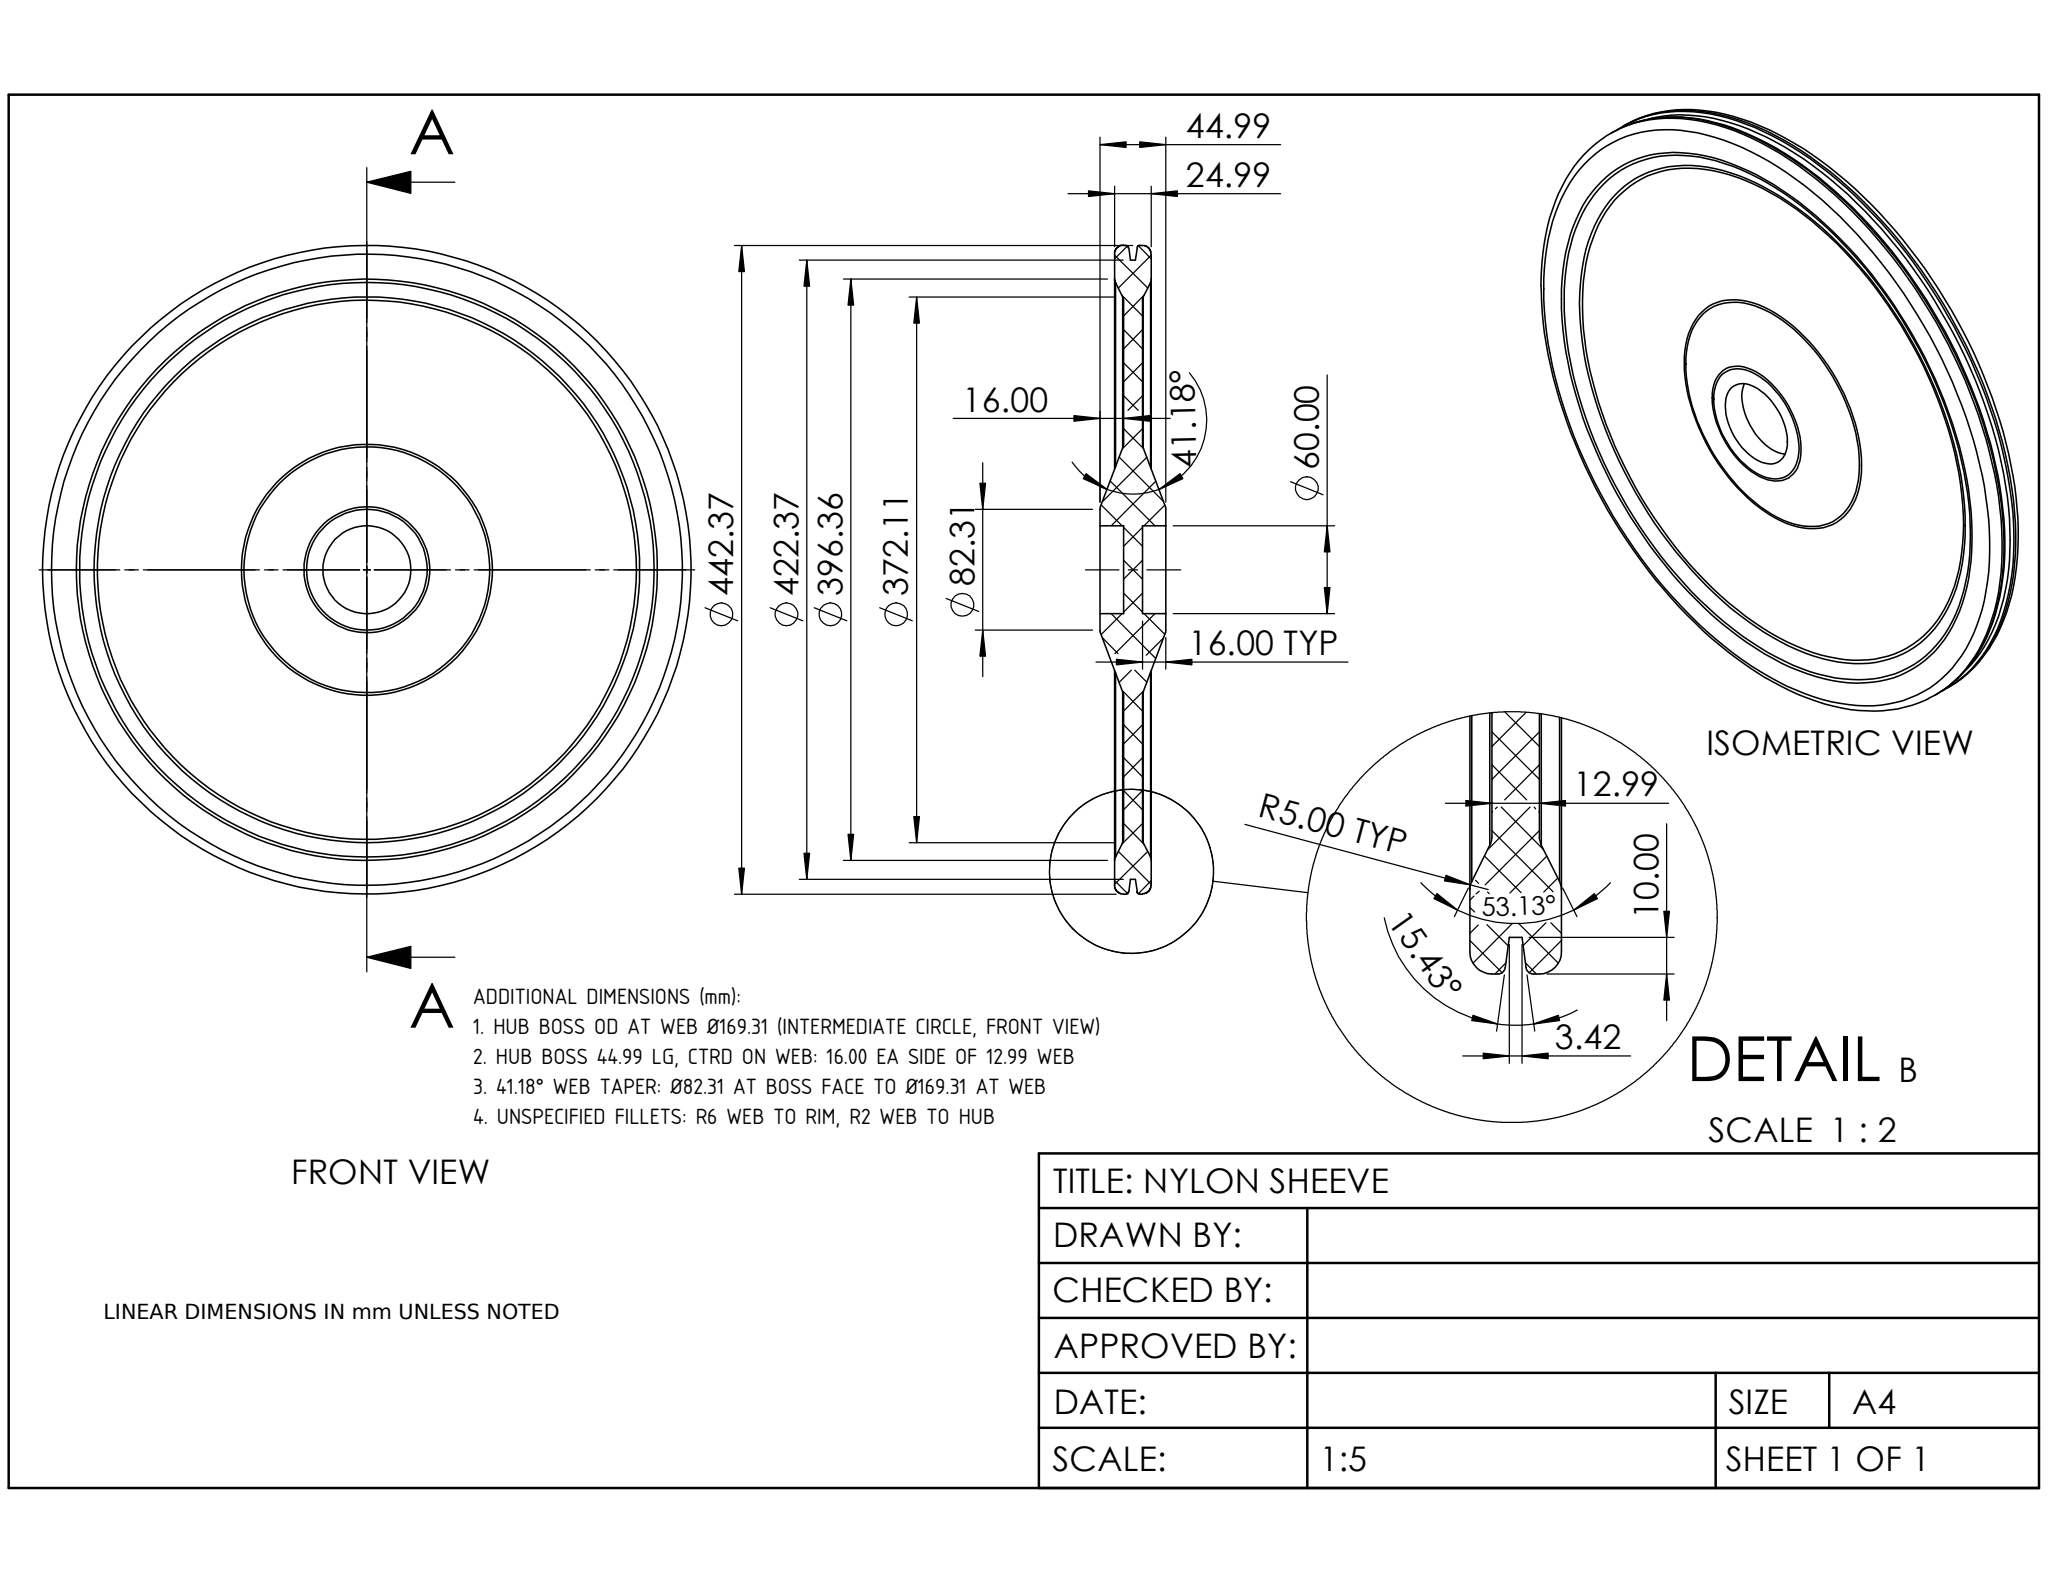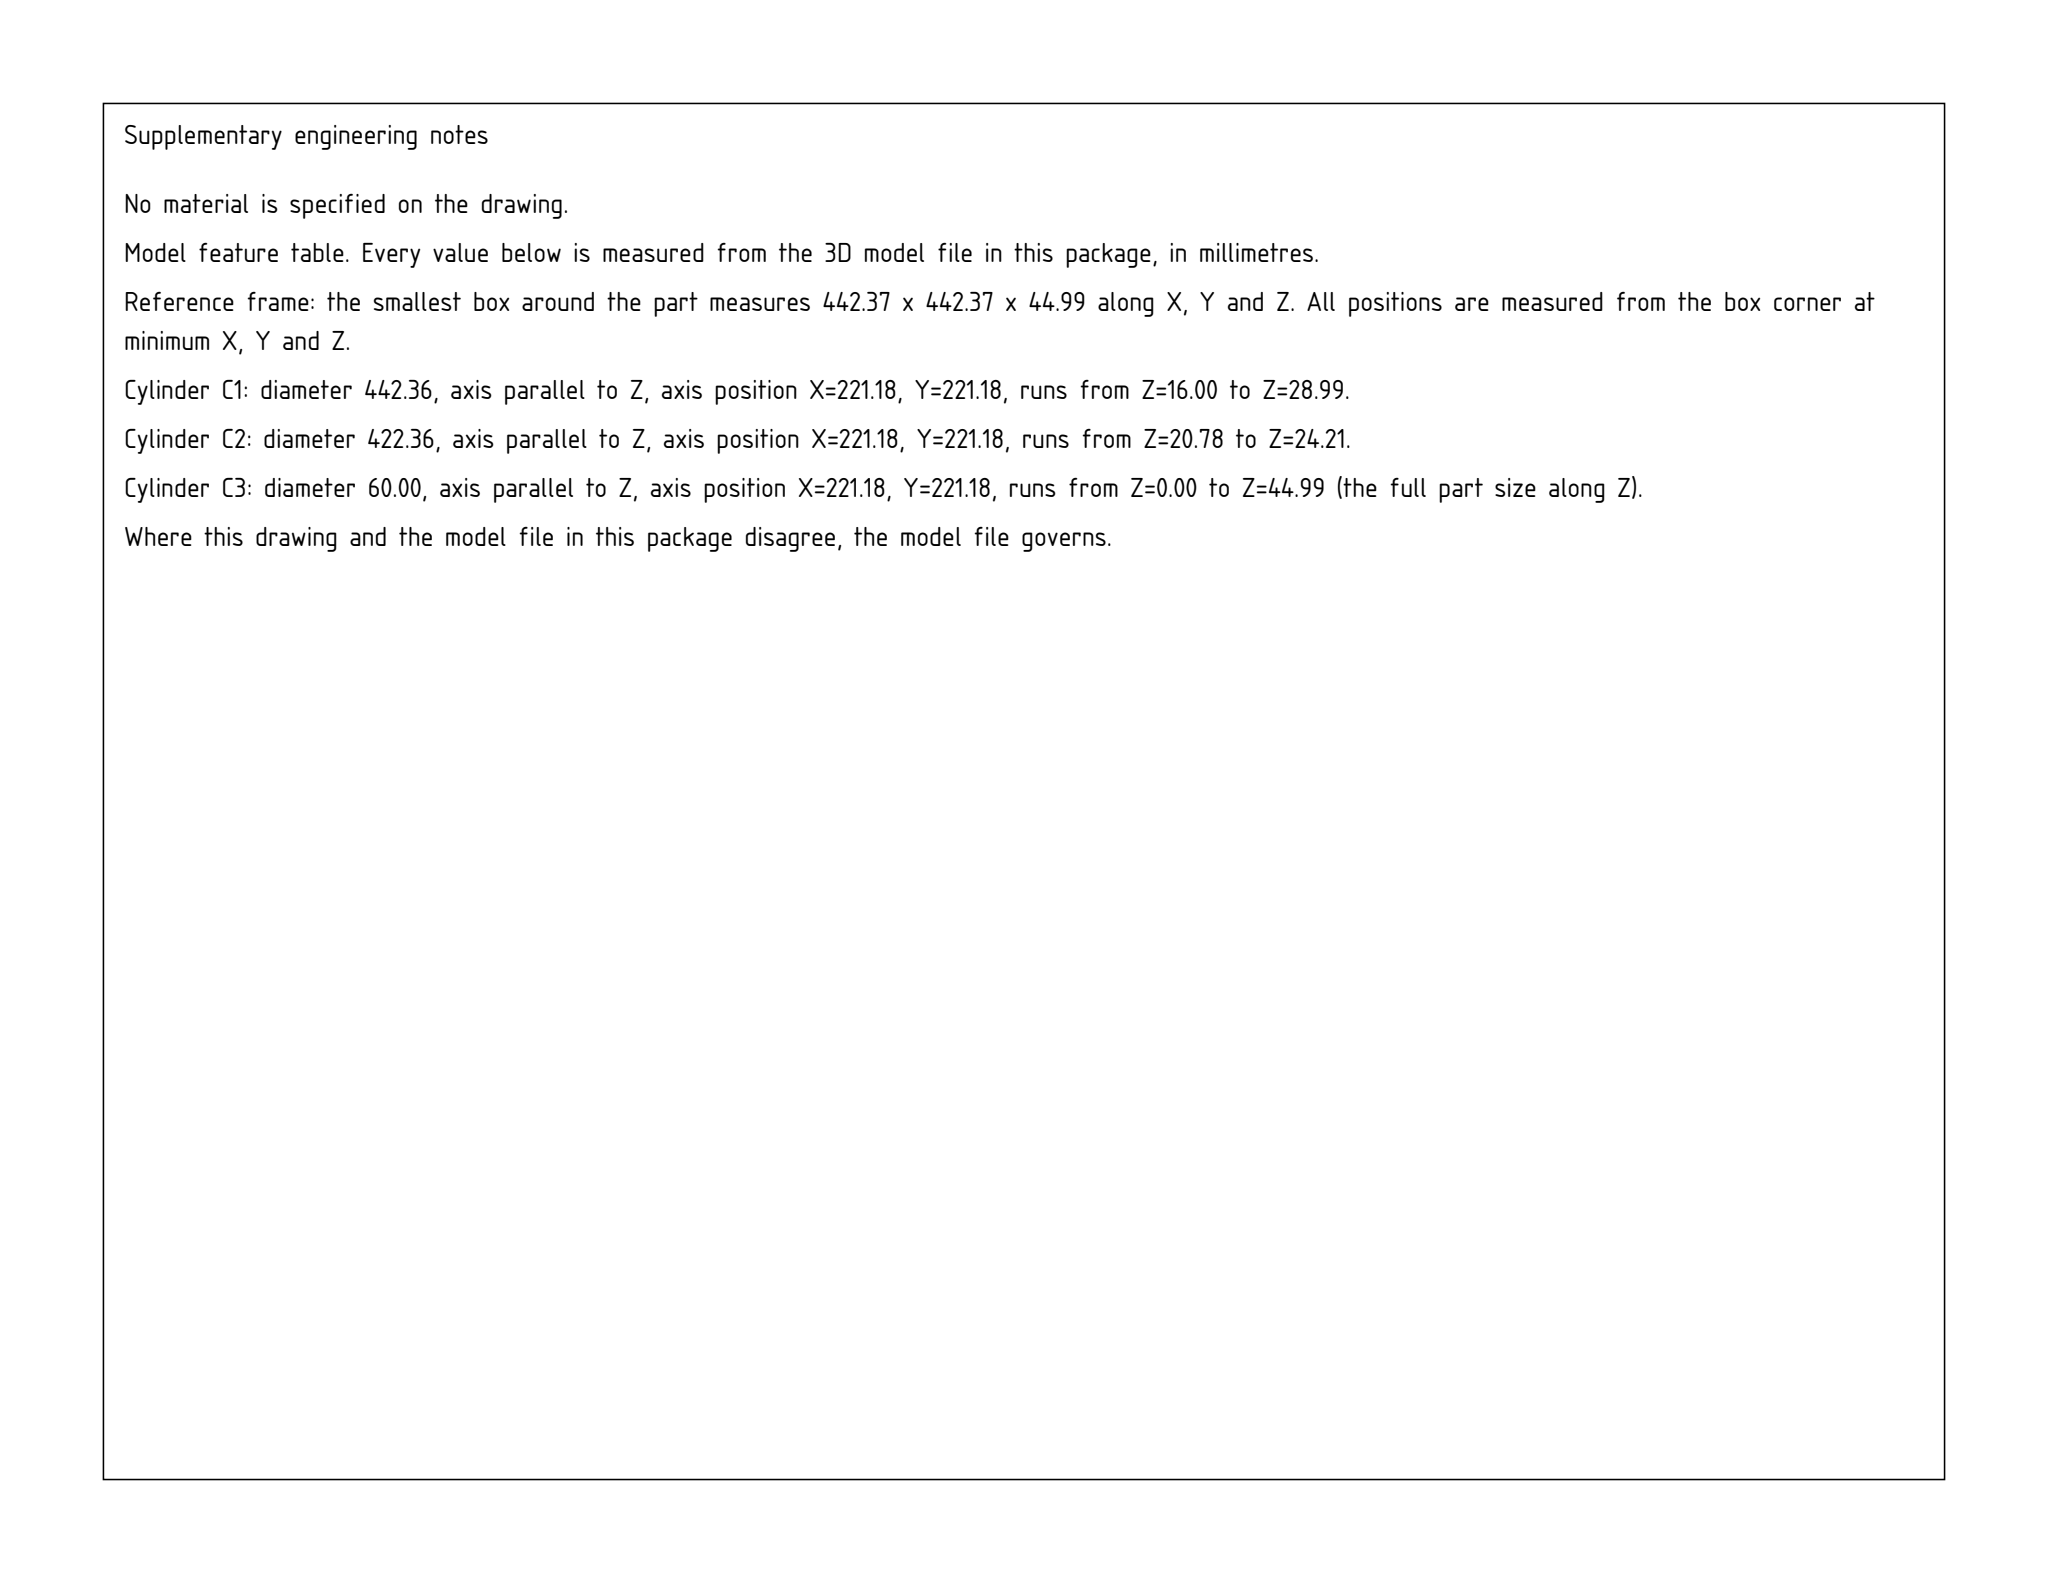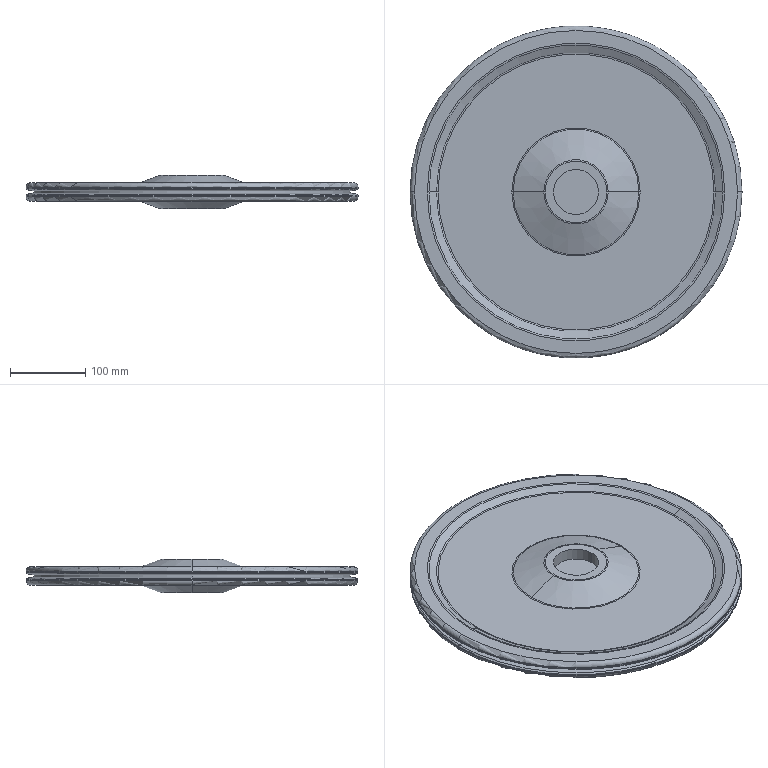Part | SolidWorks | mm | 1 solid | 54 faces | box 442.37 x 442.37 x 44.99 mm | volume 2705251 mm3 | torus 24 | cone 12 | cylinder 10 | plane 8 | commonest cylinder face diameters 60 x4 442.365 x4 422.365 x2
build123d program:
from build123d import *

# Parameters (mm, degrees)
FILLET1_R          = 6
FILLET2_R          = 2
FILLET4_R          = 5
SKETCH3_R          = 30
CUT_EXTRUDE1_DEPTH = 16


with BuildPart() as part:
    # Sketch1 → Revolve1 (revolve)
    with BuildSketch(Plane(origin=(0, 0, 0), x_dir=(0, 0, -1), z_dir=(1, 0, 0)), mode=Mode.PRIVATE) as revolve1_sk:
        Polygon((-22.495, 42.065), (-22.495, 0), (22.495, 0), (22.495, 42.065), (12.495, 89.938), (12.495, 221.183), (3.065, 221.183), (1.71, 211.183), (-1.71, 211.183), (-3.065, 221.183), (-12.495, 221.183), (-12.495, 89.938), align=None)
    revolve(revolve1_sk.sketch.rotate(Axis((0, 0, 22.495), (0, 0, -1)), 90), axis=Axis((0, 0, 22.495), (0, 0, -1)))

    # Fillet1
    fillet1_edges = [part.edges().sort_by_distance(p)[0] for p in [
        (-221.183, 0, 12.495),
        (-221.183, 0, -12.495),
    ]]
    fillet(fillet1_edges, radius=FILLET1_R)

    # Sketch2 → Cut-Revolve1 (revolve, cut)
    with BuildSketch(Plane(origin=(0, 0, 0), x_dir=(0, 0, -1), z_dir=(1, 0, 0)), mode=Mode.PRIVATE) as cut_revolve1_sk:
        Polygon((12.495, 197), (6.495, 185), (6.495, 84.655), (22.495, 42.065), (36.194, 42.065), (36.194, 126.736), (12.495, 126.736), align=None)
    cut_revolve1 = revolve(cut_revolve1_sk.sketch.rotate(Axis((0, 0, 98.304), (0, 0, -1)), 270), axis=Axis((0, 0, 98.304), (0, 0, -1)), mode=Mode.SUBTRACT)

    # Mirror3: Cut-Revolve1 across plane
    add(cut_revolve1.mirror(Plane.XY), mode=Mode.SUBTRACT)

    # Fillet2
    fillet2_edges = [part.edges().sort_by_distance(p)[0] for p in [
        (-221.183, 0, 3.065),
        (-221.183, 0, -3.065),
    ]]
    fillet(fillet2_edges, radius=FILLET2_R)

    # Fillet4
    fillet4_edges = [part.edges().sort_by_distance(p)[0] for p in [
        (197, 0, -12.495),
        (185, 0, -6.495),
        (84.655, 0, -6.495),
        (42.065, 0, -22.495),
        (197, 0, 12.495),
        (185, 0, 6.495),
        (84.655, 0, 6.495),
        (42.065, 0, 22.495),
    ]]
    fillet(fillet4_edges, radius=FILLET4_R)

    # Sketch3 → Cut-Extrude1 (cut)
    with BuildSketch(Plane.XY.offset(22.495)):
        Circle(SKETCH3_R)
    cut_extrude1 = extrude(amount=-CUT_EXTRUDE1_DEPTH, mode=Mode.SUBTRACT)

    # Mirror4: Cut-Extrude1 across plane
    add(cut_extrude1.mirror(Plane.XY), mode=Mode.SUBTRACT)


solid = part.part